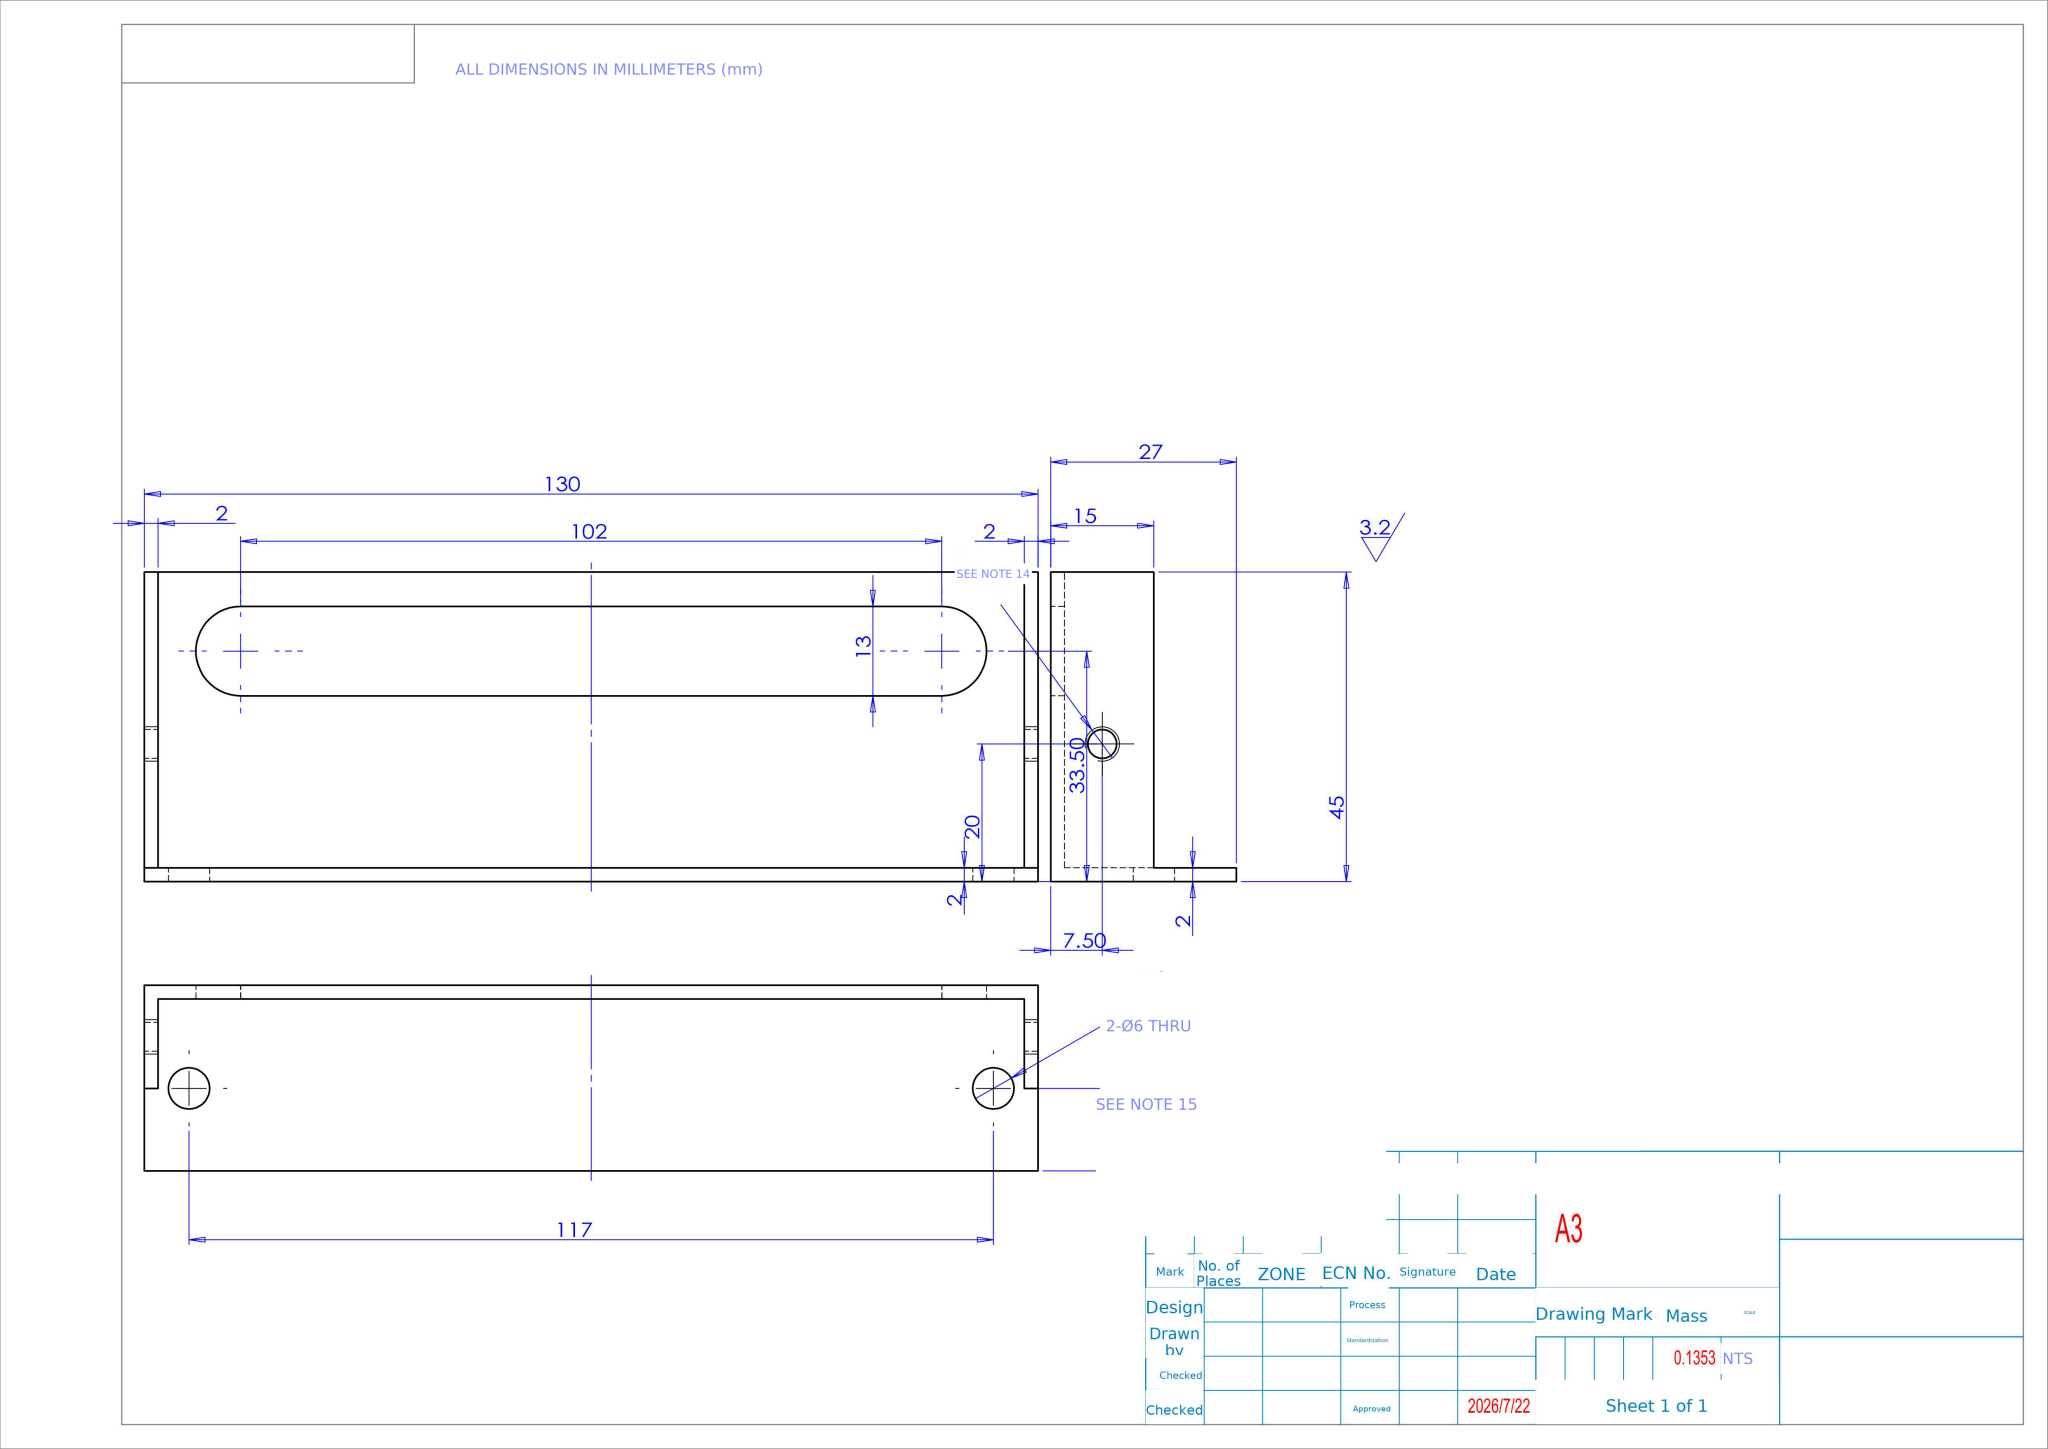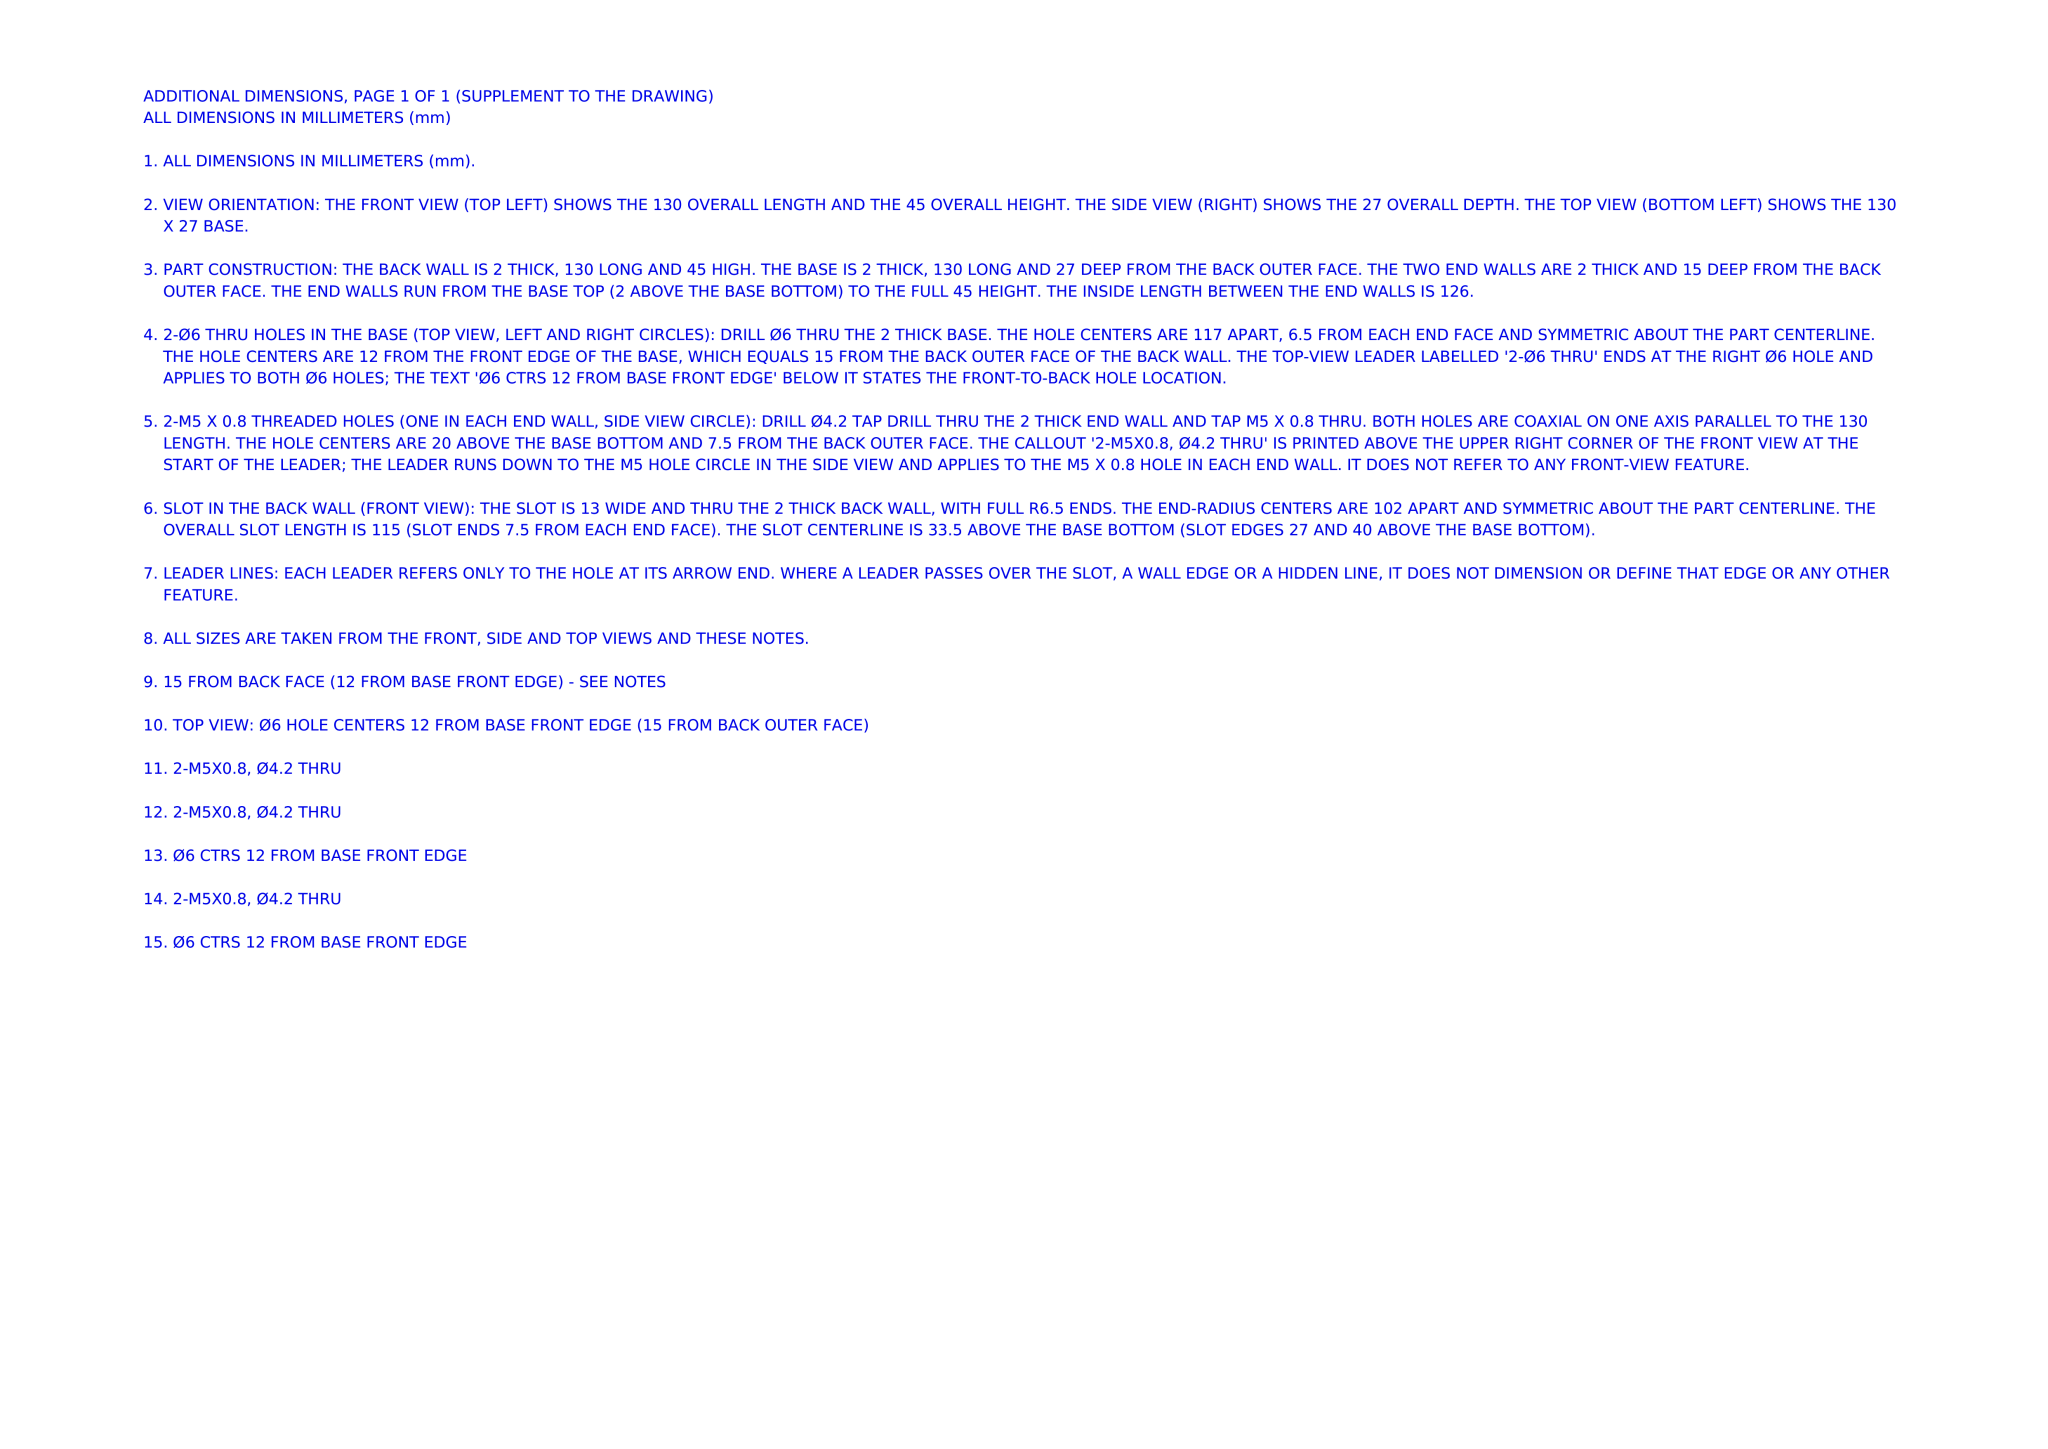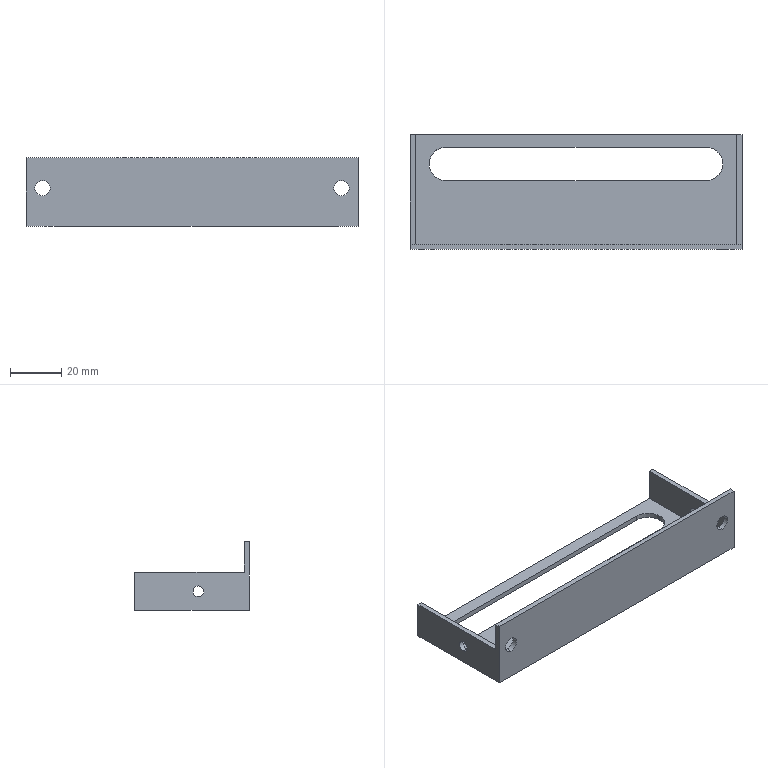Part | NX | mm | 1 solid | 25 faces | box 130 x 45 x 27 mm | volume 17350 mm3 | plane 14 | cylinder 11 | commonest cylinder face diameters 4.2 x4 6 x4 13 x3